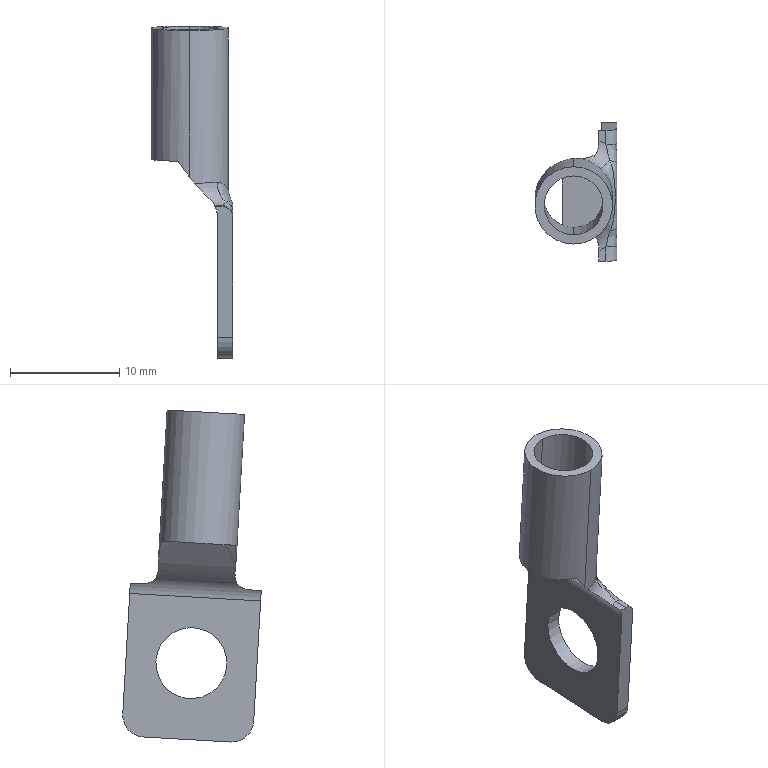Component | SolidWorks | GroundingSystem-1_SC16-6-1 | 1 solid | 28 faces | volume 456 mm3 | cylinder 11 | plane 10 | spline 5 | torus 2 | commonest cylinder face diameters 4 x3 6.5 x2 5.4 x2 7.1 x2 2 x2